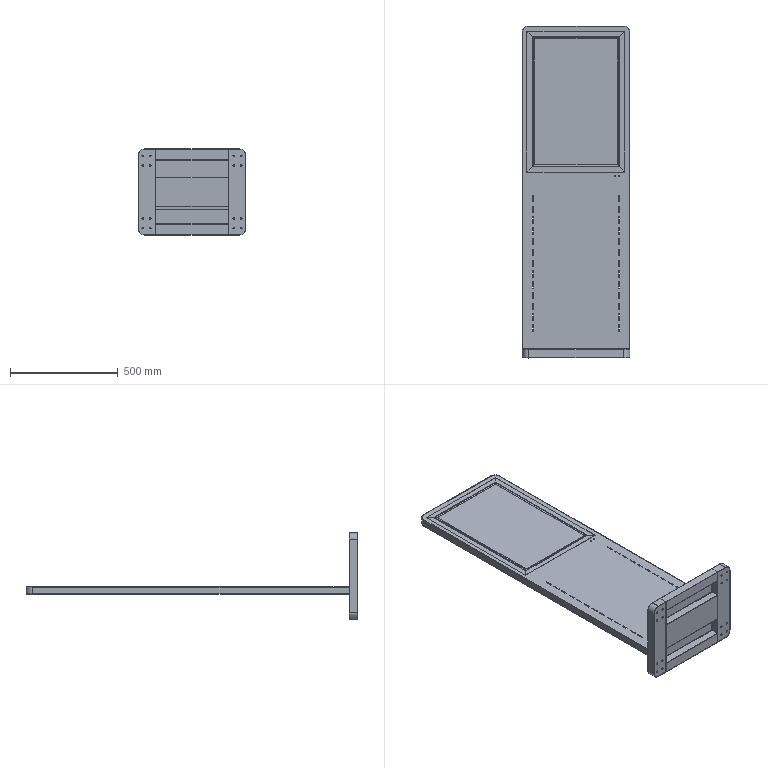Assembly | SolidWorks | mm | 21 component files | 21 solids | 646 faces | box 500 x 1540 x 400 mm | volume 2999340 mm3 | plane 464 | cylinder 174 | spline 8 | commonest cylinder face diameters 30 x42 7 x32 1 x27 4 x14 3 x13 60 x10 57 x6 2.2 x6
Bill of materials:
w7 | 2 |  | Straight thin-walled square hollow tube with both ends cut at an angle (appears mitered).
w8 | 2 |  | Straight thin-walled square hollow tube with angled (mitered) cuts at both ends; similar to unnamed part.
Mirror_Mirror_w12 | 1 |  | Thin curved shell panel with a constant-thickness quarter-circle (about 90 degree) arc section, extruded straight along its length.
Mirror_w12 | 2 |  | Thin curved shell panel with a quarter-circle arc section, extruded straight.
Mirror_w13 | 1 |  | Bent sheet angle (L-section) bracket with unequal legs, a small inside bend radius, rounded corners on one leg, and eight small through-holes in that leg in two groups of four (2x2) near each end.
w11 | 1 |  | Shallow rectangular sheet pan or cover: a flat panel with rounded corners and short bent flanges along the edges, with the flanges not meeting at the corners.
w12 | 1 |  | Thin curved shell panel with a quarter-circle arc section, extruded straight.
w13 | 1 |  | Bent sheet angle (L-section) bracket with unequal legs, a small bend radius, rounded corners on the free edge of one leg, and eight small holes in 2x2 groups near each end.
w14 | 1 |  | Formed sheet panel with a stepped (offset) profile: the section has two raised rectangular offsets, giving an alternating flat-and-offset shape, with notches at the edge ends.
Mirror_w3 | 1 |  | Thin curved shell panel with a quarter-circle arc section; it is longer along its axis relative to its arc span than the other arc panels.
Mirror_w4 | 1 |  | Flat thin plate shaped as a quarter annulus (a 90 degree ring sector), with a fairly wide radial band.
Mirror_w5 | 1 |  | Flat thin plate shaped as a quarter annulus (a 90 degree ring sector), with a narrower radial band than unnamed part.
w2 | 1 |  | Elongated rectangular flat plate with rounded corners at one end, a large rectangular through-opening occupying roughly half its length near the rounded end, and a solid remaining portion.
w3 | 1 |  | Thin-walled curved shell shaped like a quarter-cylinder segment of constant wall thickness, extruded straight along its axis.
w4 | 1 |  | Flat quarter-annulus (90-degree ring sector) plate with a relatively wide radial band and constant thickness.
w5 | 1 |  | Flat quarter-annulus (90-degree ring sector) plate with a narrower radial band than unnamed part, constant thickness.
w6 | 1 |  | Plain thin rectangular flat sheet with sharp corners and no visible holes or features.
w9 | 1 |  | Thin rectangular sheet with two rounded corners at one end and two parallel columns of ten elongated slots (twenty in total), and a narrow stepped or offset strip along the opposite edge.
Mates:
1. coincident | w2-1 face at (220, 720.75, 0) dir (0, 0, 1) | w3-1 face at (220, 720.75, 0) dir (0, 0, 1)
2. coincident | w2-1 face at (250, 720.75, -1) dir (0, 1, 0) | w3-1 face at (250, 720.75, 0) dir (0, -1, 0)
3. coincident | w2-1 face at (220, 750.75, -35) dir (1, 0, 0) | w3-1 face at (220, 749.75, 0) dir (-1, 0, 0)
4. distance | w6-1 face at (200, 98.75, -3) dir (1, 0, 0) | w2-1 face at (250, 0, 0) dir (1, 0, 0)
5. distance | w6-1 face at (200, 700.75, -3) dir (0, 1, 0) | w2-1 face at (0, 750.75, 0) dir (0, 1, 0)
6. distance | w6-1 face at (0, 399.75, -3) dir (0, 0, 1) | w2-1 face at (220, 720.75, -1) dir (0, 0, -1)
7. coincident | w2-1 face at (220, 720.75, -1) dir (0, 0, -1) | dbj2-1/w7-1 face at (-203, 72.75, -1) dir (0, 0, 1)
8. distance | dbj2-1/w8-1 face at (-228, 701.75, -1) dir (0, -1, 0) | w6-1 face at (200, 700.75, -3) dir (0, 1, 0)
9. distance | w6-1 face at (200, 98.75, -3) dir (1, 0, 0) | dbj2-1/w7-2 face at (201, 726.75, -1) dir (-1, 0, 0)
10. coincident | w2-1 face at (0, 0, -33.7) dir (0, 0, -1) | w9-1 face at (-219.5, 720.25, -33.7) dir (0, 0, 1)
11. distance | w9-1 face at (-219.5, 742.25, -33.7) dir (0, 1, 0) | w2-1 face at (0, 742.75, 0) dir (0, -1, 0)
12. distance | w9-1 face at (241.5, 42.25, -33.7) dir (1, 0, 0) | w2-1 face at (242, 0, 0) dir (-1, 0, 0)
13. coincident | w2-1 face at (0, -749.25, 0) dir (0, -1, 0) | dbj3-1/w11-1 face at (-220, -749.25, 220) dir (0, 1, 0)
14. coincident | w2-1 face at (250, 0, 0) dir (1, 0, 0) | dbj3-1/w11-1 face at (250, -749.25, 50) dir (1, 0, 0)
15. distance | w2-1 face at (220, 720.75, 0) dir (0, 0, 1) | dbj3-1/w11-1 face at (0, -749.25, 250) dir (0, 0, 1)
16. coincident | w7-1 face at (23.847, -18.622, 354) dir (1, 0, 0) | w8-2 face at (23.847, -447.622, 329) dir (1, 0, 0)
17. coincident | w7-1 face at (873.791, 6.378, 354) dir (0, -0.7071, 0.7071) | w8-2 face at (624.316, 6.378, 354) dir (0, 0.7071, -0.7071)
18. coincident | w7-1 face at (23.847, -18.622, 354) dir (1, 0, 0) | w8-1 face at (23.847, 6.378, -275) dir (1, 0, 0)
19. coincident | w7-1 face at (873.791, 6.378, -300) dir (0, -0.7071, -0.7071) | w8-1 face at (624.316, 6.378, -300) dir (0, 0.7071, 0.7071)
20. coincident | w7-1 edge at (23.847, 6.378, -300) dir (-1, 0, 0) | w8-1 edge at (23.847, 6.378, -300) dir (-1, 0, 0)
21. coincident | w7-1 edge at (23.847, 6.378, 354) dir (-1, 0, 0) | w8-2 edge at (23.847, 6.378, 354) dir (-1, 0, 0)
22. coincident | w7-1 face at (23.847, -18.622, 354) dir (1, 0, 0) | w7-2 face at (23.847, -422.622, -300) dir (1, 0, 0)
23. coincident | w7-2 face at (873.791, -447.622, 354) dir (0, 0.7071, 0.7071) | w8-2 face at (624.316, -447.622, 354) dir (0, -0.7071, -0.7071)
24. coincident | w7-2 edge at (23.847, -447.622, 354) dir (-1, 0, 0) | w8-2 edge at (23.847, -447.622, 354) dir (-1, 0, 0)
25. coincident | w11-1 face at (-220.896, -168.358, 20) dir (0, 0, 1) | w12-1 face at (219.104, 171.642, 20) dir (0, 0, 1)
26. coincident | w11-1 face at (249.104, 171.642, 18.5) dir (0, 1, 0) | w12-1 face at (249.104, 171.642, 20) dir (0, -1, 0)
27. coincident | w11-1 face at (219.104, 201.642, -20) dir (1, 0, 0) | w12-1 face at (219.104, 200.142, 20) dir (-1, 0, 0)
28. coincident | w11-1 face at (247.604, 1.642, 20) dir (-1, 0, 0) | w13-1 face at (247.604, -196.358, -18.5) dir (1, 0, 0)
29. coincident | w11-1 face at (-220.896, -168.358, 18.5) dir (0, 0, -1) | w13-1 face at (167.604, -196.358, 18.5) dir (0, 0, 1)
30. distance | w13-1 face at (169.604, 199.642, -18) dir (0, 1, 0) | w11-1 face at (-0.8959, 200.142, 20) dir (0, -1, 0)
31. coincident | w11-1 face at (-220.896, -168.358, 18.5) dir (0, 0, -1) | w14-1 face at (167.604, -66.858, 18.5) dir (0, 0, 1)
32. coincident | w13-1 face at (167.604, -196.358, -20) dir (-1, 0, 0) | w14-1 face at (167.604, -64.858, -18.5) dir (1, 0, 0)
33. coincident | w11-1 face at (-0.8959, 200.142, 20) dir (0, -1, 0) | w14-1 face at (167.604, 200.142, -18.5) dir (0, 1, 0)